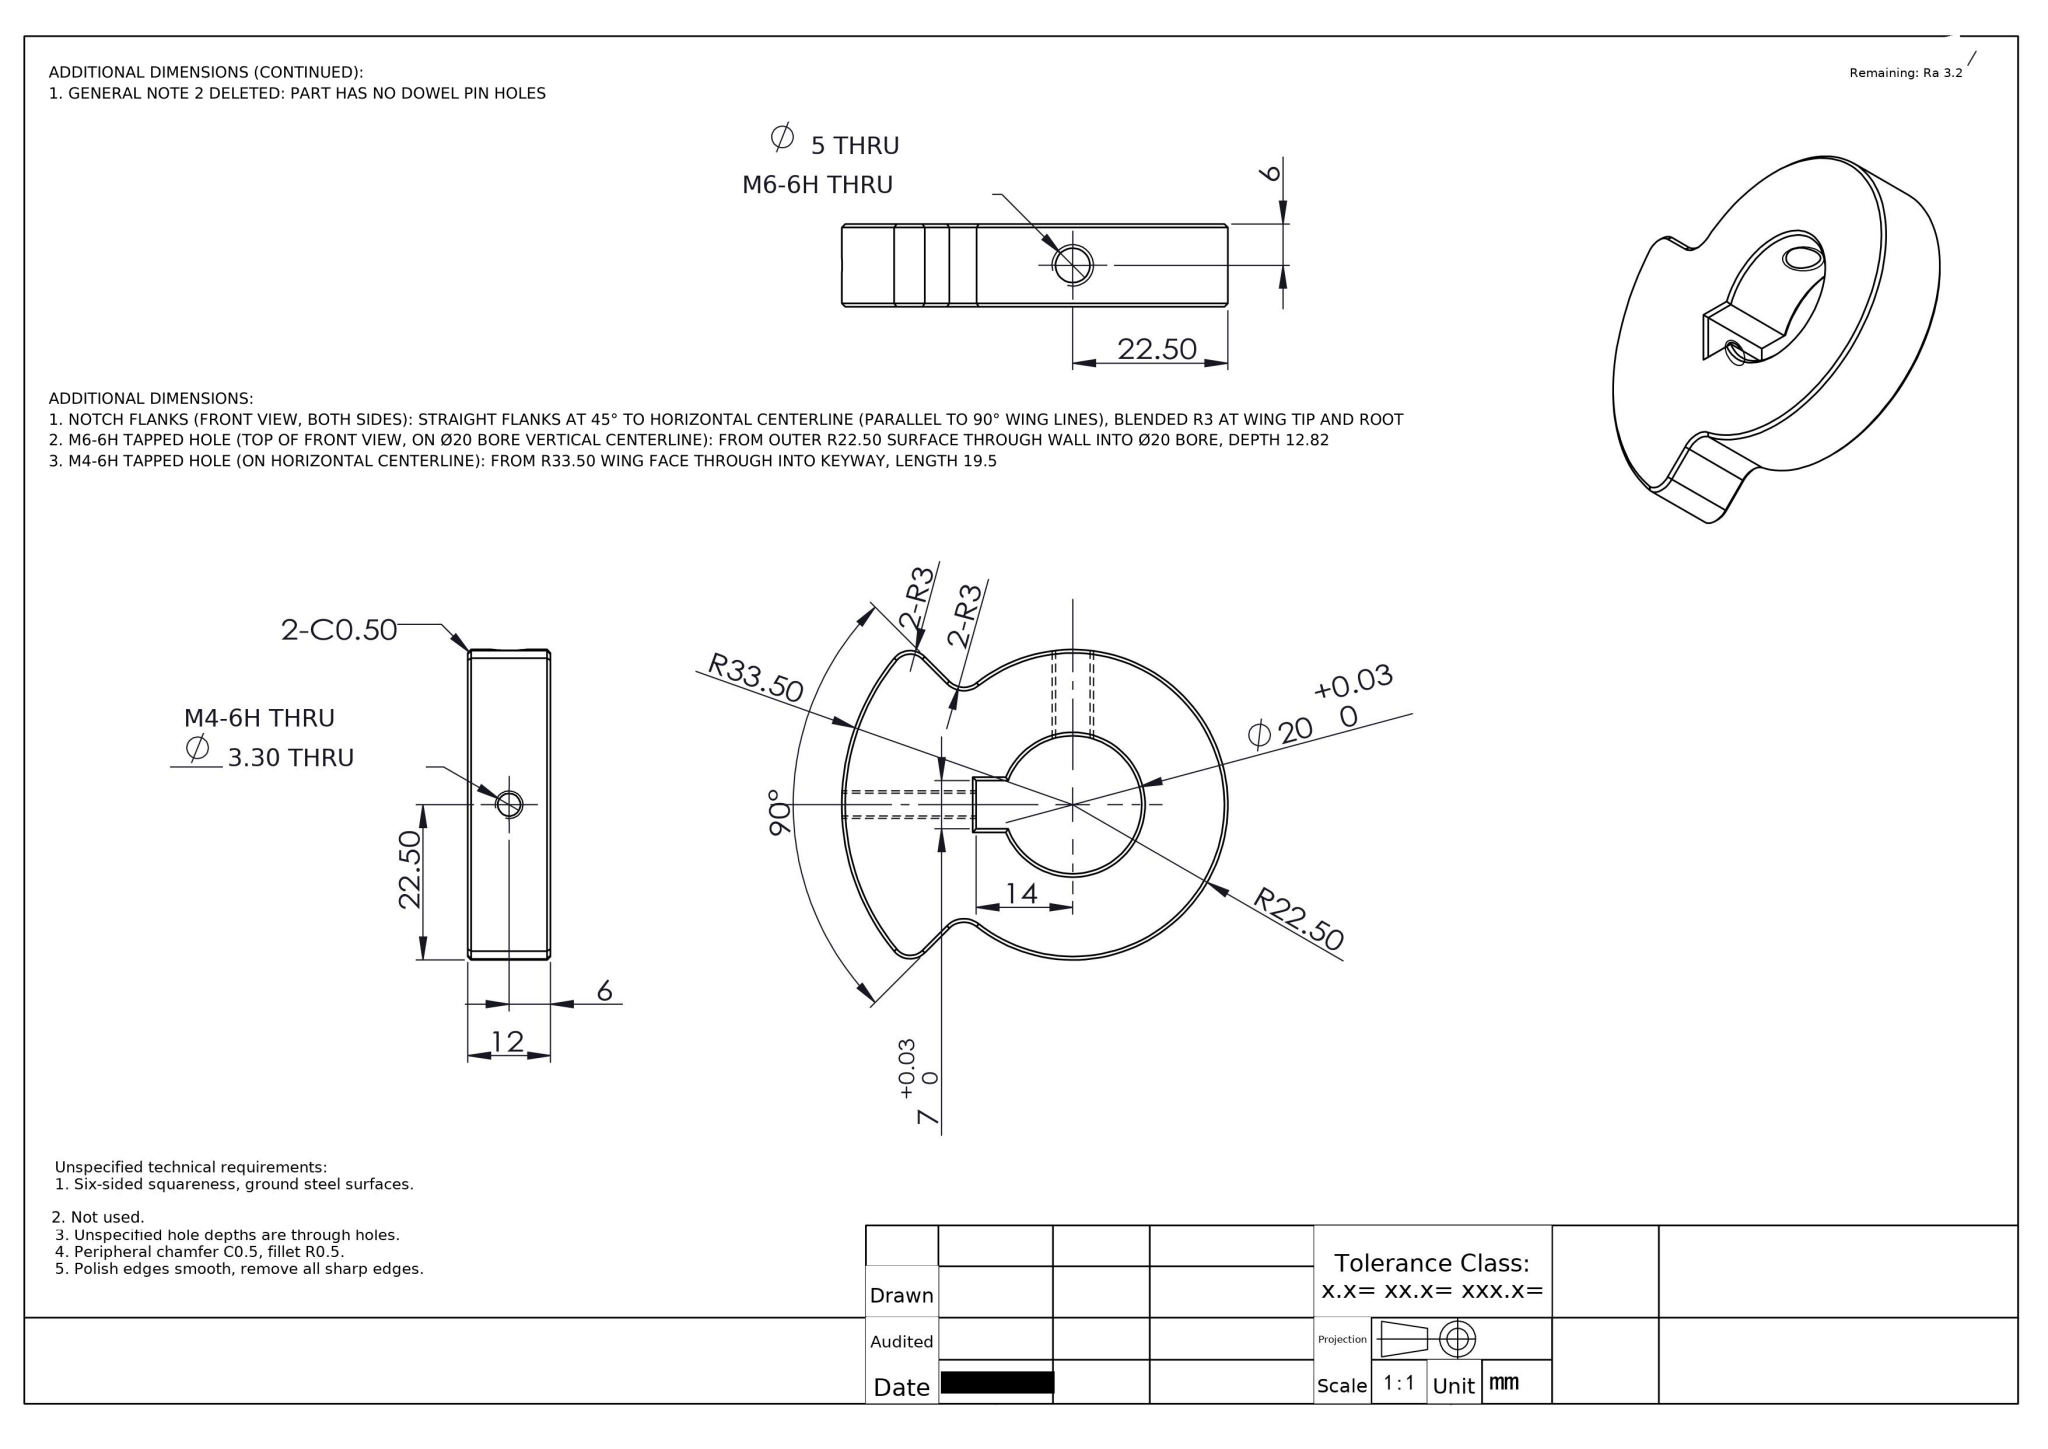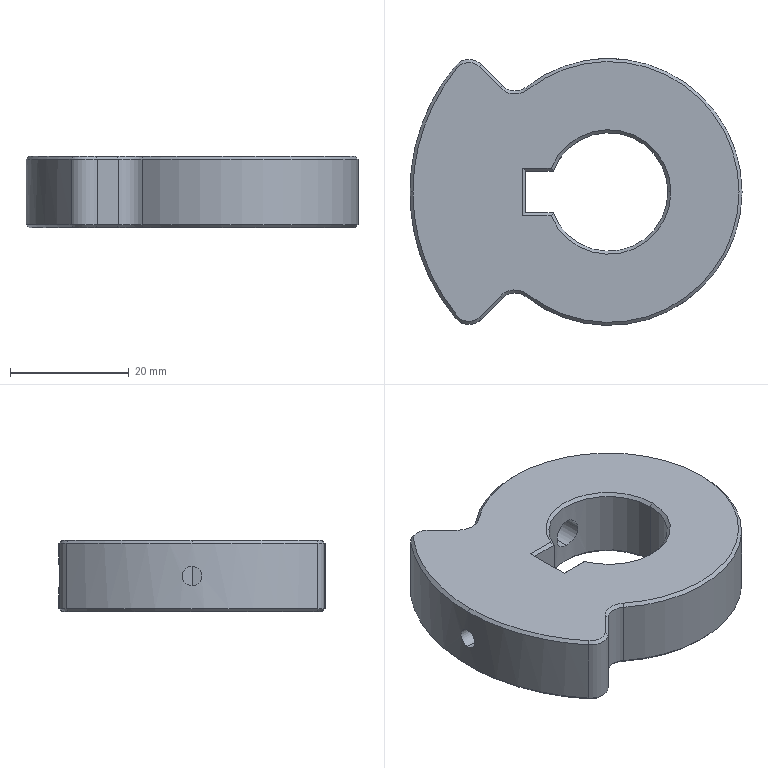Part | NX | mm | 1 solid | 47 faces | box 56 x 45 x 12 mm | volume 20277 mm3 | cone 17 | plane 17 | cylinder 13 | commonest cylinder face diameters 6 x4 3.3 x2 5 x2 45 x2 20 x2 67 x1